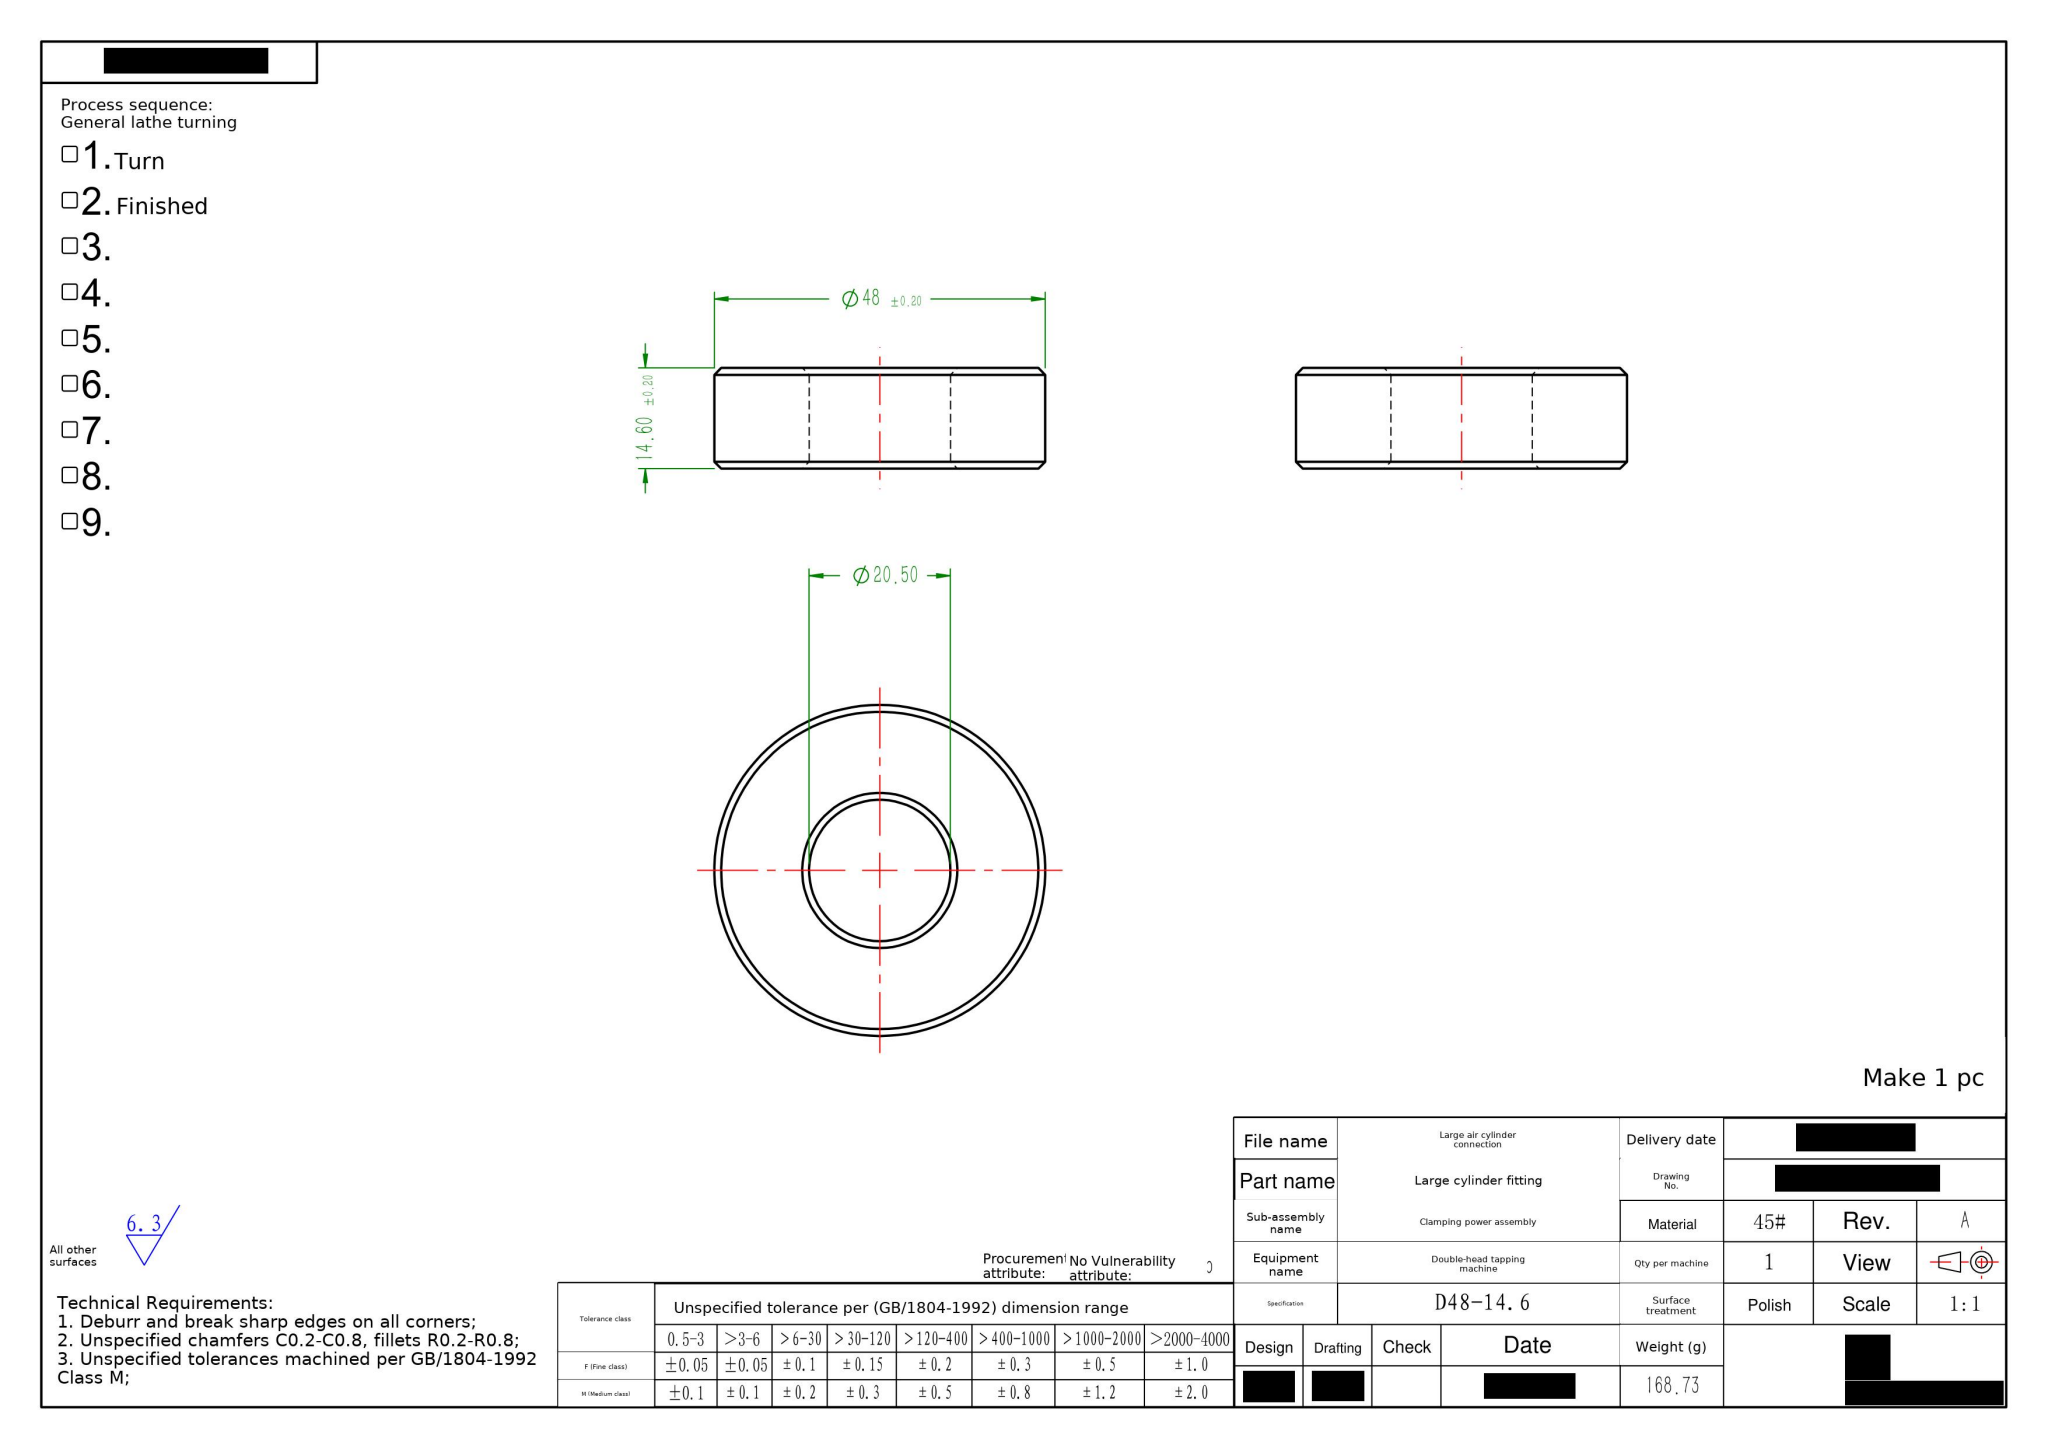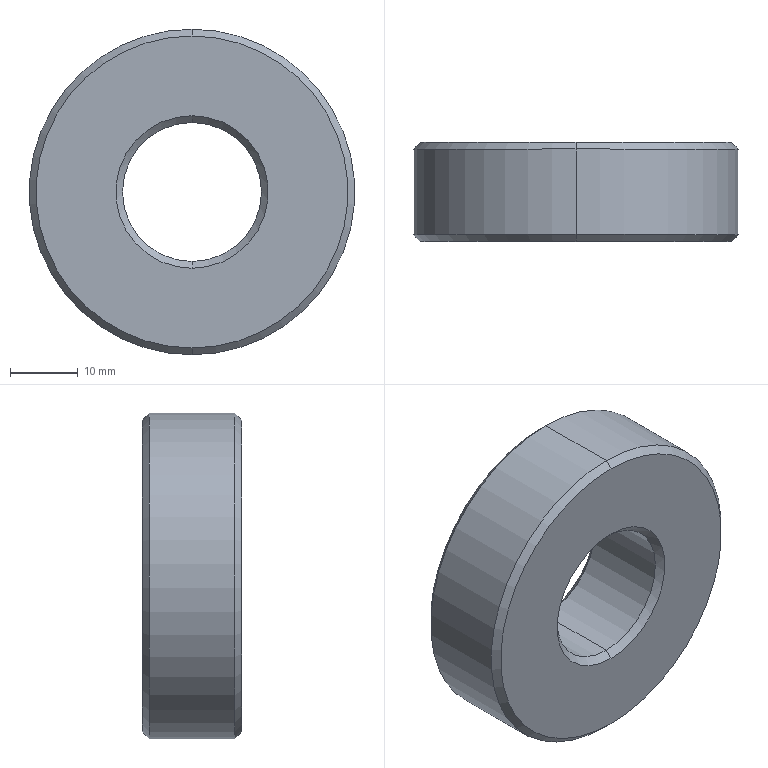Part | SolidWorks | mm | material 45# | 1 solid | 14 faces | box 48 x 14.6 x 48 mm | volume 21385 mm3 | cone 8 | cylinder 4 | plane 2 | commonest cylinder face diameters 20.5 x2 48 x2
build123d program:
from build123d import *

# Parameters (mm, degrees)
SKETCH1_R           = 24
SKETCH1_R_2         = 10.25
BOSS_EXTRUDE1_DEPTH = 14.6
CHAMFER1_SIZE       = 1


with BuildPart() as part:
    # Sketch1 → Boss-Extrude1 (new body)
    with BuildSketch(Plane(origin=(0, 0, 0), x_dir=(1, 0, 0), z_dir=(0, 1, 0))):
        with Locations(Location((0, 0, 0), (0, 0, 270))):
            Circle(SKETCH1_R)
        with Locations(Location((0, 0, 0), (0, 0, 270))):
            Circle(SKETCH1_R_2, mode=Mode.SUBTRACT)
    extrude(amount=BOSS_EXTRUDE1_DEPTH)

    # Chamfer1
    chamfer1_edges = [part.edges().sort_by_distance(p)[0] for p in [
        (0, 0, -24),
        (0, 14.6, -24),
        (0, 0, -10.25),
        (0, 14.6, -10.25),
    ]]
    chamfer(chamfer1_edges, length=CHAMFER1_SIZE)


solid = part.part
STEP:
#1=CARTESIAN_POINT('',(0.,13.6,-10.25));
#2=VERTEX_POINT('',#1);
#3=CARTESIAN_POINT('',(0.,13.6,10.25));
#4=VERTEX_POINT('',#3);
#5=CARTESIAN_POINT('',(0.,13.6,0.));
#6=DIRECTION('',(0.,1.,0.));
#7=DIRECTION('',(0.,0.,1.));
#8=AXIS2_PLACEMENT_3D('',#5,#6,#7);
#9=CIRCLE('',#8,10.25);
#10=EDGE_CURVE('',#2,#4,#9,.T.);
#11=ORIENTED_EDGE('',*,*,#10,.F.);
#12=CARTESIAN_POINT('',(0.,14.6,-11.25));
#13=VERTEX_POINT('',#12);
#14=CARTESIAN_POINT('',(0.,13.6,-10.25));
#15=DIRECTION('',(0.,0.7071,-0.7071));
#16=VECTOR('',#15,1000.);
#17=LINE('',#14,#16);
#18=EDGE_CURVE('',#2,#13,#17,.T.);
#19=ORIENTED_EDGE('',*,*,#18,.T.);
#20=CARTESIAN_POINT('',(0.,14.6,11.25));
#21=VERTEX_POINT('',#20);
#22=CARTESIAN_POINT('',(0.,14.6,0.));
#23=DIRECTION('',(0.,-1.,0.));
#24=DIRECTION('',(0.,0.,1.));
#25=AXIS2_PLACEMENT_3D('',#22,#23,#24);
#26=CIRCLE('',#25,11.25);
#27=EDGE_CURVE('',#21,#13,#26,.T.);
#28=ORIENTED_EDGE('',*,*,#27,.F.);
#29=CARTESIAN_POINT('',(0.,13.6,10.25));
#30=DIRECTION('',(0.,0.7071,0.7071));
#31=VECTOR('',#30,1000.);
#32=LINE('',#29,#31);
#33=EDGE_CURVE('',#4,#21,#32,.T.);
#34=ORIENTED_EDGE('',*,*,#33,.F.);
#35=EDGE_LOOP('',(#11,#19,#28,#34));
#36=FACE_OUTER_BOUND('',#35,.T.);
#37=CARTESIAN_POINT('',(0.,13.6,0.));
#38=DIRECTION('',(0.,1.,0.));
#39=DIRECTION('',(0.,0.,1.));
#40=AXIS2_PLACEMENT_3D('',#37,#38,#39);
#41=CONICAL_SURFACE('',#40,10.25,0.7854);
#42=ADVANCED_FACE('',(#36),#41,.F.);
#43=CARTESIAN_POINT('',(0.,1.,10.25));
#44=VERTEX_POINT('',#43);
#45=CARTESIAN_POINT('',(0.,1.,-10.25));
#46=VERTEX_POINT('',#45);
#47=CARTESIAN_POINT('',(0.,1.,0.));
#48=DIRECTION('',(0.,-1.,0.));
#49=DIRECTION('',(0.,0.,1.));
#50=AXIS2_PLACEMENT_3D('',#47,#48,#49);
#51=CIRCLE('',#50,10.25);
#52=EDGE_CURVE('',#44,#46,#51,.T.);
#53=ORIENTED_EDGE('',*,*,#52,.F.);
#54=CARTESIAN_POINT('',(0.,0.,11.25));
#55=VERTEX_POINT('',#54);
#56=CARTESIAN_POINT('',(0.,0.,11.25));
#57=DIRECTION('',(0.,-0.7071,0.7071));
#58=VECTOR('',#57,1000.);
#59=LINE('',#56,#58);
#60=EDGE_CURVE('',#44,#55,#59,.T.);
#61=ORIENTED_EDGE('',*,*,#60,.T.);
#62=CARTESIAN_POINT('',(0.,0.,-11.25));
#63=VERTEX_POINT('',#62);
#64=CARTESIAN_POINT('',(0.,0.,0.));
#65=DIRECTION('',(0.,1.,0.));
#66=DIRECTION('',(0.,0.,1.));
#67=AXIS2_PLACEMENT_3D('',#64,#65,#66);
#68=CIRCLE('',#67,11.25);
#69=EDGE_CURVE('',#63,#55,#68,.T.);
#70=ORIENTED_EDGE('',*,*,#69,.F.);
#71=CARTESIAN_POINT('',(0.,0.,-11.25));
#72=DIRECTION('',(0.,-0.7071,-0.7071));
#73=VECTOR('',#72,1000.);
#74=LINE('',#71,#73);
#75=EDGE_CURVE('',#46,#63,#74,.T.);
#76=ORIENTED_EDGE('',*,*,#75,.F.);
#77=EDGE_LOOP('',(#53,#61,#70,#76));
#78=FACE_OUTER_BOUND('',#77,.T.);
#79=CARTESIAN_POINT('',(0.,0.,0.));
#80=DIRECTION('',(0.,-1.,0.));
#81=DIRECTION('',(0.,0.,-1.));
#82=AXIS2_PLACEMENT_3D('',#79,#80,#81);
#83=CONICAL_SURFACE('',#82,11.25,0.7854);
#84=ADVANCED_FACE('',(#78),#83,.F.);
#85=CARTESIAN_POINT('',(0.,14.6,23.));
#86=VERTEX_POINT('',#85);
#87=CARTESIAN_POINT('',(0.,14.6,-23.));
#88=VERTEX_POINT('',#87);
#89=CARTESIAN_POINT('',(0.,14.6,0.));
#90=DIRECTION('',(0.,1.,0.));
#91=DIRECTION('',(0.,0.,1.));
#92=AXIS2_PLACEMENT_3D('',#89,#90,#91);
#93=CIRCLE('',#92,23.);
#94=EDGE_CURVE('',#86,#88,#93,.T.);
#95=ORIENTED_EDGE('',*,*,#94,.F.);
#96=CARTESIAN_POINT('',(0.,13.6,24.));
#97=VERTEX_POINT('',#96);
#98=CARTESIAN_POINT('',(0.,14.6,23.));
#99=DIRECTION('',(0.,-0.7071,0.7071));
#100=VECTOR('',#99,1000.);
#101=LINE('',#98,#100);
#102=EDGE_CURVE('',#86,#97,#101,.T.);
#103=ORIENTED_EDGE('',*,*,#102,.T.);
#104=CARTESIAN_POINT('',(0.,13.6,-24.));
#105=VERTEX_POINT('',#104);
#106=CARTESIAN_POINT('',(0.,13.6,0.));
#107=DIRECTION('',(0.,-1.,0.));
#108=DIRECTION('',(0.,0.,1.));
#109=AXIS2_PLACEMENT_3D('',#106,#107,#108);
#110=CIRCLE('',#109,24.);
#111=EDGE_CURVE('',#105,#97,#110,.T.);
#112=ORIENTED_EDGE('',*,*,#111,.F.);
#113=CARTESIAN_POINT('',(0.,14.6,-23.));
#114=DIRECTION('',(0.,-0.7071,-0.7071));
#115=VECTOR('',#114,1000.);
#116=LINE('',#113,#115);
#117=EDGE_CURVE('',#88,#105,#116,.T.);
#118=ORIENTED_EDGE('',*,*,#117,.F.);
#119=EDGE_LOOP('',(#95,#103,#112,#118));
#120=FACE_OUTER_BOUND('',#119,.T.);
#121=CARTESIAN_POINT('',(0.,14.6,0.));
#122=DIRECTION('',(0.,-1.,0.));
#123=DIRECTION('',(0.,0.,-1.));
#124=AXIS2_PLACEMENT_3D('',#121,#122,#123);
#125=CONICAL_SURFACE('',#124,23.,0.7854);
#126=ADVANCED_FACE('',(#120),#125,.T.);
#127=CARTESIAN_POINT('',(0.,0.,-23.));
#128=VERTEX_POINT('',#127);
#129=CARTESIAN_POINT('',(0.,0.,23.));
#130=VERTEX_POINT('',#129);
#131=CARTESIAN_POINT('',(0.,0.,0.));
#132=DIRECTION('',(0.,-1.,0.));
#133=DIRECTION('',(0.,0.,1.));
#134=AXIS2_PLACEMENT_3D('',#131,#132,#133);
#135=CIRCLE('',#134,23.);
#136=EDGE_CURVE('',#128,#130,#135,.T.);
#137=ORIENTED_EDGE('',*,*,#136,.F.);
#138=CARTESIAN_POINT('',(0.,1.,-24.));
#139=VERTEX_POINT('',#138);
#140=CARTESIAN_POINT('',(0.,1.,-24.));
#141=DIRECTION('',(0.,0.7071,-0.7071));
#142=VECTOR('',#141,1000.);
#143=LINE('',#140,#142);
#144=EDGE_CURVE('',#128,#139,#143,.T.);
#145=ORIENTED_EDGE('',*,*,#144,.T.);
#146=CARTESIAN_POINT('',(0.,1.,24.));
#147=VERTEX_POINT('',#146);
#148=CARTESIAN_POINT('',(0.,1.,0.));
#149=DIRECTION('',(0.,1.,0.));
#150=DIRECTION('',(0.,0.,1.));
#151=AXIS2_PLACEMENT_3D('',#148,#149,#150);
#152=CIRCLE('',#151,24.);
#153=EDGE_CURVE('',#147,#139,#152,.T.);
#154=ORIENTED_EDGE('',*,*,#153,.F.);
#155=CARTESIAN_POINT('',(0.,1.,24.));
#156=DIRECTION('',(0.,0.7071,0.7071));
#157=VECTOR('',#156,1000.);
#158=LINE('',#155,#157);
#159=EDGE_CURVE('',#130,#147,#158,.T.);
#160=ORIENTED_EDGE('',*,*,#159,.F.);
#161=EDGE_LOOP('',(#137,#145,#154,#160));
#162=FACE_OUTER_BOUND('',#161,.T.);
#163=CARTESIAN_POINT('',(0.,1.,0.));
#164=DIRECTION('',(0.,1.,0.));
#165=DIRECTION('',(0.,0.,1.));
#166=AXIS2_PLACEMENT_3D('',#163,#164,#165);
#167=CONICAL_SURFACE('',#166,24.,0.7854);
#168=ADVANCED_FACE('',(#162),#167,.T.);
#169=ORIENTED_EDGE('',*,*,#10,.T.);
#170=CARTESIAN_POINT('',(0.,14.6,10.25));
#171=DIRECTION('',(0.,-1.,0.));
#172=VECTOR('',#171,1000.);
#173=LINE('',#170,#172);
#174=EDGE_CURVE('',#4,#44,#173,.T.);
#175=ORIENTED_EDGE('',*,*,#174,.T.);
#176=ORIENTED_EDGE('',*,*,#52,.T.);
#177=CARTESIAN_POINT('',(0.,14.6,-10.25));
#178=DIRECTION('',(0.,-1.,0.));
#179=VECTOR('',#178,1000.);
#180=LINE('',#177,#179);
#181=EDGE_CURVE('',#2,#46,#180,.T.);
#182=ORIENTED_EDGE('',*,*,#181,.F.);
#183=EDGE_LOOP('',(#169,#175,#176,#182));
#184=FACE_OUTER_BOUND('',#183,.T.);
#185=CARTESIAN_POINT('',(0.,14.6,0.));
#186=DIRECTION('',(0.,-1.,0.));
#187=DIRECTION('',(0.,0.,-1.));
#188=AXIS2_PLACEMENT_3D('',#185,#186,#187);
#189=CYLINDRICAL_SURFACE('',#188,10.25);
#190=ADVANCED_FACE('',(#184),#189,.F.);
#191=ORIENTED_EDGE('',*,*,#111,.T.);
#192=CARTESIAN_POINT('',(0.,14.6,24.));
#193=DIRECTION('',(0.,-1.,0.));
#194=VECTOR('',#193,1000.);
#195=LINE('',#192,#194);
#196=EDGE_CURVE('',#97,#147,#195,.T.);
#197=ORIENTED_EDGE('',*,*,#196,.T.);
#198=ORIENTED_EDGE('',*,*,#153,.T.);
#199=CARTESIAN_POINT('',(0.,14.6,-24.));
#200=DIRECTION('',(0.,-1.,0.));
#201=VECTOR('',#200,1000.);
#202=LINE('',#199,#201);
#203=EDGE_CURVE('',#105,#139,#202,.T.);
#204=ORIENTED_EDGE('',*,*,#203,.F.);
#205=EDGE_LOOP('',(#191,#197,#198,#204));
#206=FACE_OUTER_BOUND('',#205,.T.);
#207=CARTESIAN_POINT('',(0.,14.6,0.));
#208=DIRECTION('',(0.,-1.,0.));
#209=DIRECTION('',(0.,0.,-1.));
#210=AXIS2_PLACEMENT_3D('',#207,#208,#209);
#211=CYLINDRICAL_SURFACE('',#210,24.);
#212=ADVANCED_FACE('',(#206),#211,.T.);
#213=CARTESIAN_POINT('',(0.,14.6,0.));
#214=DIRECTION('',(0.,1.,0.));
#215=DIRECTION('',(0.,0.,1.));
#216=AXIS2_PLACEMENT_3D('',#213,#214,#215);
#217=CIRCLE('',#216,23.);
#218=EDGE_CURVE('',#88,#86,#217,.T.);
#219=ORIENTED_EDGE('',*,*,#218,.T.);
#220=ORIENTED_EDGE('',*,*,#94,.T.);
#221=EDGE_LOOP('',(#219,#220));
#222=FACE_OUTER_BOUND('',#221,.T.);
#223=ORIENTED_EDGE('',*,*,#27,.T.);
#224=CARTESIAN_POINT('',(0.,14.6,0.));
#225=DIRECTION('',(0.,-1.,0.));
#226=DIRECTION('',(0.,0.,1.));
#227=AXIS2_PLACEMENT_3D('',#224,#225,#226);
#228=CIRCLE('',#227,11.25);
#229=EDGE_CURVE('',#13,#21,#228,.T.);
#230=ORIENTED_EDGE('',*,*,#229,.T.);
#231=EDGE_LOOP('',(#223,#230));
#232=FACE_BOUND('',#231,.T.);
#233=CARTESIAN_POINT('',(0.,14.6,0.));
#234=DIRECTION('',(0.,1.,0.));
#235=DIRECTION('',(0.,0.,1.));
#236=AXIS2_PLACEMENT_3D('',#233,#234,#235);
#237=PLANE('',#236);
#238=ADVANCED_FACE('',(#222,#232),#237,.T.);
#239=CARTESIAN_POINT('',(0.,0.,0.));
#240=DIRECTION('',(0.,-1.,0.));
#241=DIRECTION('',(0.,0.,1.));
#242=AXIS2_PLACEMENT_3D('',#239,#240,#241);
#243=CIRCLE('',#242,23.);
#244=EDGE_CURVE('',#130,#128,#243,.T.);
#245=ORIENTED_EDGE('',*,*,#244,.T.);
#246=ORIENTED_EDGE('',*,*,#136,.T.);
#247=EDGE_LOOP('',(#245,#246));
#248=FACE_OUTER_BOUND('',#247,.T.);
#249=ORIENTED_EDGE('',*,*,#69,.T.);
#250=CARTESIAN_POINT('',(0.,0.,0.));
#251=DIRECTION('',(0.,1.,0.));
#252=DIRECTION('',(0.,0.,1.));
#253=AXIS2_PLACEMENT_3D('',#250,#251,#252);
#254=CIRCLE('',#253,11.25);
#255=EDGE_CURVE('',#55,#63,#254,.T.);
#256=ORIENTED_EDGE('',*,*,#255,.T.);
#257=EDGE_LOOP('',(#249,#256));
#258=FACE_BOUND('',#257,.T.);
#259=CARTESIAN_POINT('',(0.,0.,0.));
#260=DIRECTION('',(0.,1.,0.));
#261=DIRECTION('',(0.,0.,1.));
#262=AXIS2_PLACEMENT_3D('',#259,#260,#261);
#263=PLANE('',#262);
#264=ADVANCED_FACE('',(#248,#258),#263,.F.);
#265=ORIENTED_EDGE('',*,*,#196,.F.);
#266=CARTESIAN_POINT('',(0.,13.6,0.));
#267=DIRECTION('',(0.,-1.,0.));
#268=DIRECTION('',(0.,0.,1.));
#269=AXIS2_PLACEMENT_3D('',#266,#267,#268);
#270=CIRCLE('',#269,24.);
#271=EDGE_CURVE('',#97,#105,#270,.T.);
#272=ORIENTED_EDGE('',*,*,#271,.T.);
#273=ORIENTED_EDGE('',*,*,#203,.T.);
#274=CARTESIAN_POINT('',(0.,1.,0.));
#275=DIRECTION('',(0.,1.,0.));
#276=DIRECTION('',(0.,0.,1.));
#277=AXIS2_PLACEMENT_3D('',#274,#275,#276);
#278=CIRCLE('',#277,24.);
#279=EDGE_CURVE('',#139,#147,#278,.T.);
#280=ORIENTED_EDGE('',*,*,#279,.T.);
#281=EDGE_LOOP('',(#265,#272,#273,#280));
#282=FACE_OUTER_BOUND('',#281,.T.);
#283=CARTESIAN_POINT('',(0.,14.6,0.));
#284=DIRECTION('',(0.,-1.,0.));
#285=DIRECTION('',(0.,0.,-1.));
#286=AXIS2_PLACEMENT_3D('',#283,#284,#285);
#287=CYLINDRICAL_SURFACE('',#286,24.);
#288=ADVANCED_FACE('',(#282),#287,.T.);
#289=ORIENTED_EDGE('',*,*,#174,.F.);
#290=CARTESIAN_POINT('',(0.,13.6,0.));
#291=DIRECTION('',(0.,1.,0.));
#292=DIRECTION('',(0.,0.,1.));
#293=AXIS2_PLACEMENT_3D('',#290,#291,#292);
#294=CIRCLE('',#293,10.25);
#295=EDGE_CURVE('',#4,#2,#294,.T.);
#296=ORIENTED_EDGE('',*,*,#295,.T.);
#297=ORIENTED_EDGE('',*,*,#181,.T.);
#298=CARTESIAN_POINT('',(0.,1.,0.));
#299=DIRECTION('',(0.,-1.,0.));
#300=DIRECTION('',(0.,0.,1.));
#301=AXIS2_PLACEMENT_3D('',#298,#299,#300);
#302=CIRCLE('',#301,10.25);
#303=EDGE_CURVE('',#46,#44,#302,.T.);
#304=ORIENTED_EDGE('',*,*,#303,.T.);
#305=EDGE_LOOP('',(#289,#296,#297,#304));
#306=FACE_OUTER_BOUND('',#305,.T.);
#307=CARTESIAN_POINT('',(0.,14.6,0.));
#308=DIRECTION('',(0.,-1.,0.));
#309=DIRECTION('',(0.,0.,-1.));
#310=AXIS2_PLACEMENT_3D('',#307,#308,#309);
#311=CYLINDRICAL_SURFACE('',#310,10.25);
#312=ADVANCED_FACE('',(#306),#311,.F.);
#313=ORIENTED_EDGE('',*,*,#144,.F.);
#314=ORIENTED_EDGE('',*,*,#244,.F.);
#315=ORIENTED_EDGE('',*,*,#159,.T.);
#316=ORIENTED_EDGE('',*,*,#279,.F.);
#317=EDGE_LOOP('',(#313,#314,#315,#316));
#318=FACE_OUTER_BOUND('',#317,.T.);
#319=CARTESIAN_POINT('',(0.,1.,0.));
#320=DIRECTION('',(0.,1.,0.));
#321=DIRECTION('',(0.,0.,1.));
#322=AXIS2_PLACEMENT_3D('',#319,#320,#321);
#323=CONICAL_SURFACE('',#322,24.,0.7854);
#324=ADVANCED_FACE('',(#318),#323,.T.);
#325=ORIENTED_EDGE('',*,*,#102,.F.);
#326=ORIENTED_EDGE('',*,*,#218,.F.);
#327=ORIENTED_EDGE('',*,*,#117,.T.);
#328=ORIENTED_EDGE('',*,*,#271,.F.);
#329=EDGE_LOOP('',(#325,#326,#327,#328));
#330=FACE_OUTER_BOUND('',#329,.T.);
#331=CARTESIAN_POINT('',(0.,14.6,0.));
#332=DIRECTION('',(0.,-1.,0.));
#333=DIRECTION('',(0.,0.,-1.));
#334=AXIS2_PLACEMENT_3D('',#331,#332,#333);
#335=CONICAL_SURFACE('',#334,23.,0.7854);
#336=ADVANCED_FACE('',(#330),#335,.T.);
#337=ORIENTED_EDGE('',*,*,#60,.F.);
#338=ORIENTED_EDGE('',*,*,#303,.F.);
#339=ORIENTED_EDGE('',*,*,#75,.T.);
#340=ORIENTED_EDGE('',*,*,#255,.F.);
#341=EDGE_LOOP('',(#337,#338,#339,#340));
#342=FACE_OUTER_BOUND('',#341,.T.);
#343=CARTESIAN_POINT('',(0.,0.,0.));
#344=DIRECTION('',(0.,-1.,0.));
#345=DIRECTION('',(0.,0.,-1.));
#346=AXIS2_PLACEMENT_3D('',#343,#344,#345);
#347=CONICAL_SURFACE('',#346,11.25,0.7854);
#348=ADVANCED_FACE('',(#342),#347,.F.);
#349=ORIENTED_EDGE('',*,*,#18,.F.);
#350=ORIENTED_EDGE('',*,*,#295,.F.);
#351=ORIENTED_EDGE('',*,*,#33,.T.);
#352=ORIENTED_EDGE('',*,*,#229,.F.);
#353=EDGE_LOOP('',(#349,#350,#351,#352));
#354=FACE_OUTER_BOUND('',#353,.T.);
#355=CARTESIAN_POINT('',(0.,13.6,0.));
#356=DIRECTION('',(0.,1.,0.));
#357=DIRECTION('',(0.,0.,1.));
#358=AXIS2_PLACEMENT_3D('',#355,#356,#357);
#359=CONICAL_SURFACE('',#358,10.25,0.7854);
#360=ADVANCED_FACE('',(#354),#359,.F.);
#361=CLOSED_SHELL('',(#42,#84,#126,#168,#190,#212,#238,#264,#288,#312,#324,#336,#348,#360));
#362=MANIFOLD_SOLID_BREP('',#361);
#363=CARTESIAN_POINT('',(0.,0.,0.));
#364=DIRECTION('',(0.,0.,1.));
#365=DIRECTION('',(1.,0.,0.));
#366=AXIS2_PLACEMENT_3D('',#363,#364,#365);
#367=(LENGTH_UNIT()NAMED_UNIT(*)SI_UNIT(.MILLI.,.METRE.));
#368=UNCERTAINTY_MEASURE_WITH_UNIT(LENGTH_MEASURE(0.00001),#367,'','');
#369=(NAMED_UNIT(*)PLANE_ANGLE_UNIT()SI_UNIT($,.RADIAN.));
#370=(NAMED_UNIT(*)SI_UNIT($,.STERADIAN.)SOLID_ANGLE_UNIT());
#371=(GEOMETRIC_REPRESENTATION_CONTEXT(3)GLOBAL_UNCERTAINTY_ASSIGNED_CONTEXT((#368))GLOBAL_UNIT_ASSIGNED_CONTEXT((#367,#369,#370))REPRESENTATION_CONTEXT('',''));
#372=ADVANCED_BREP_SHAPE_REPRESENTATION('',(#362,#366),#371);